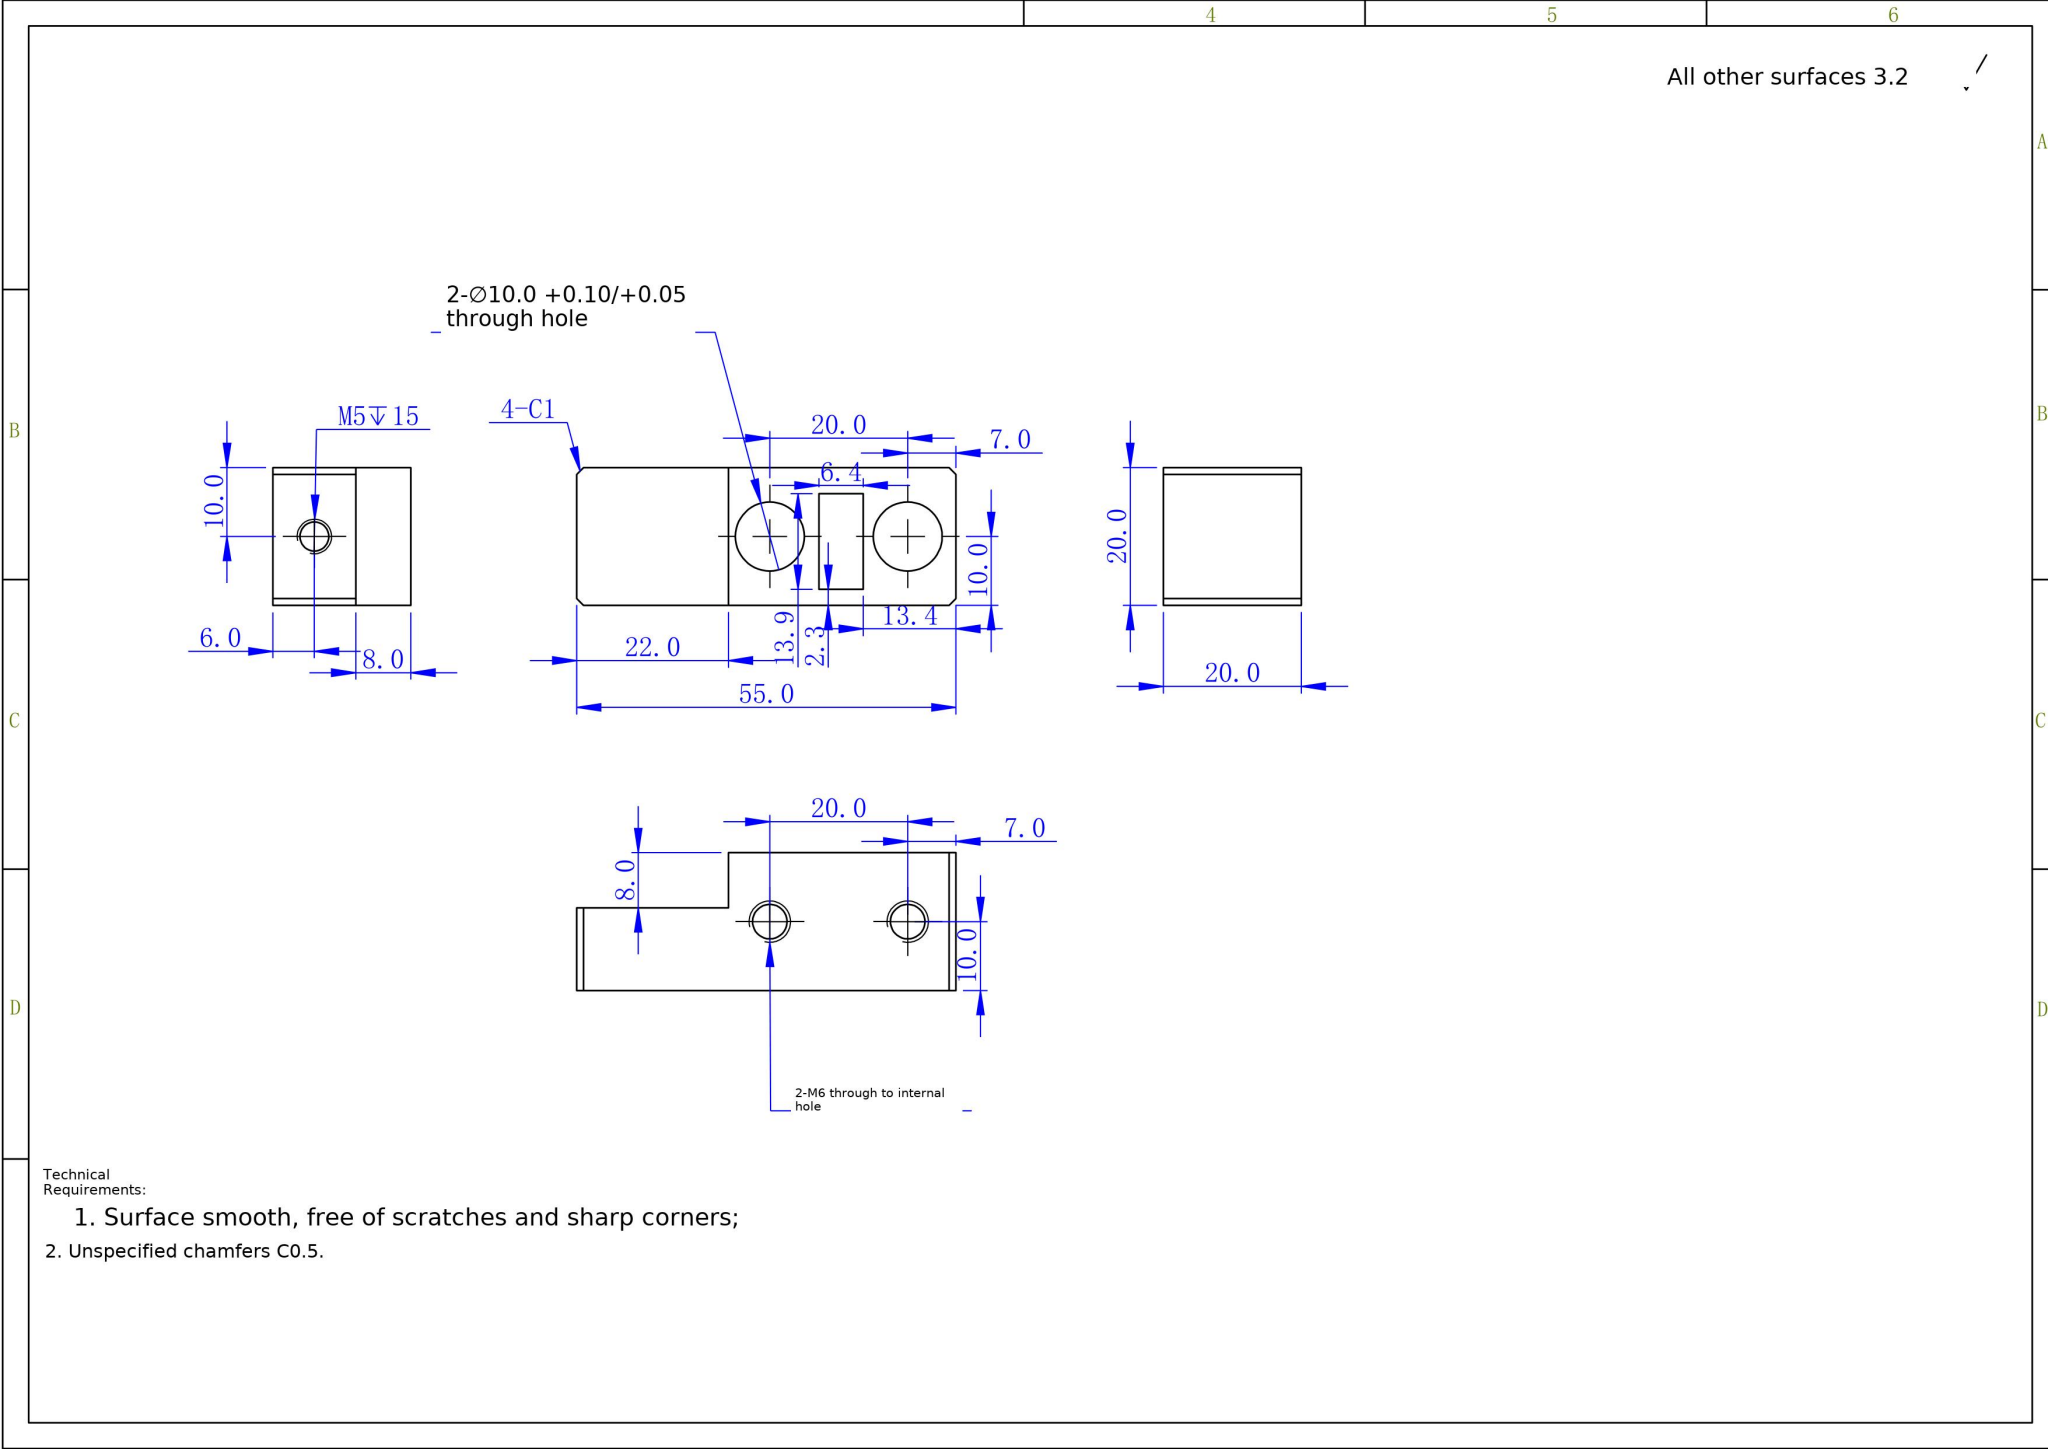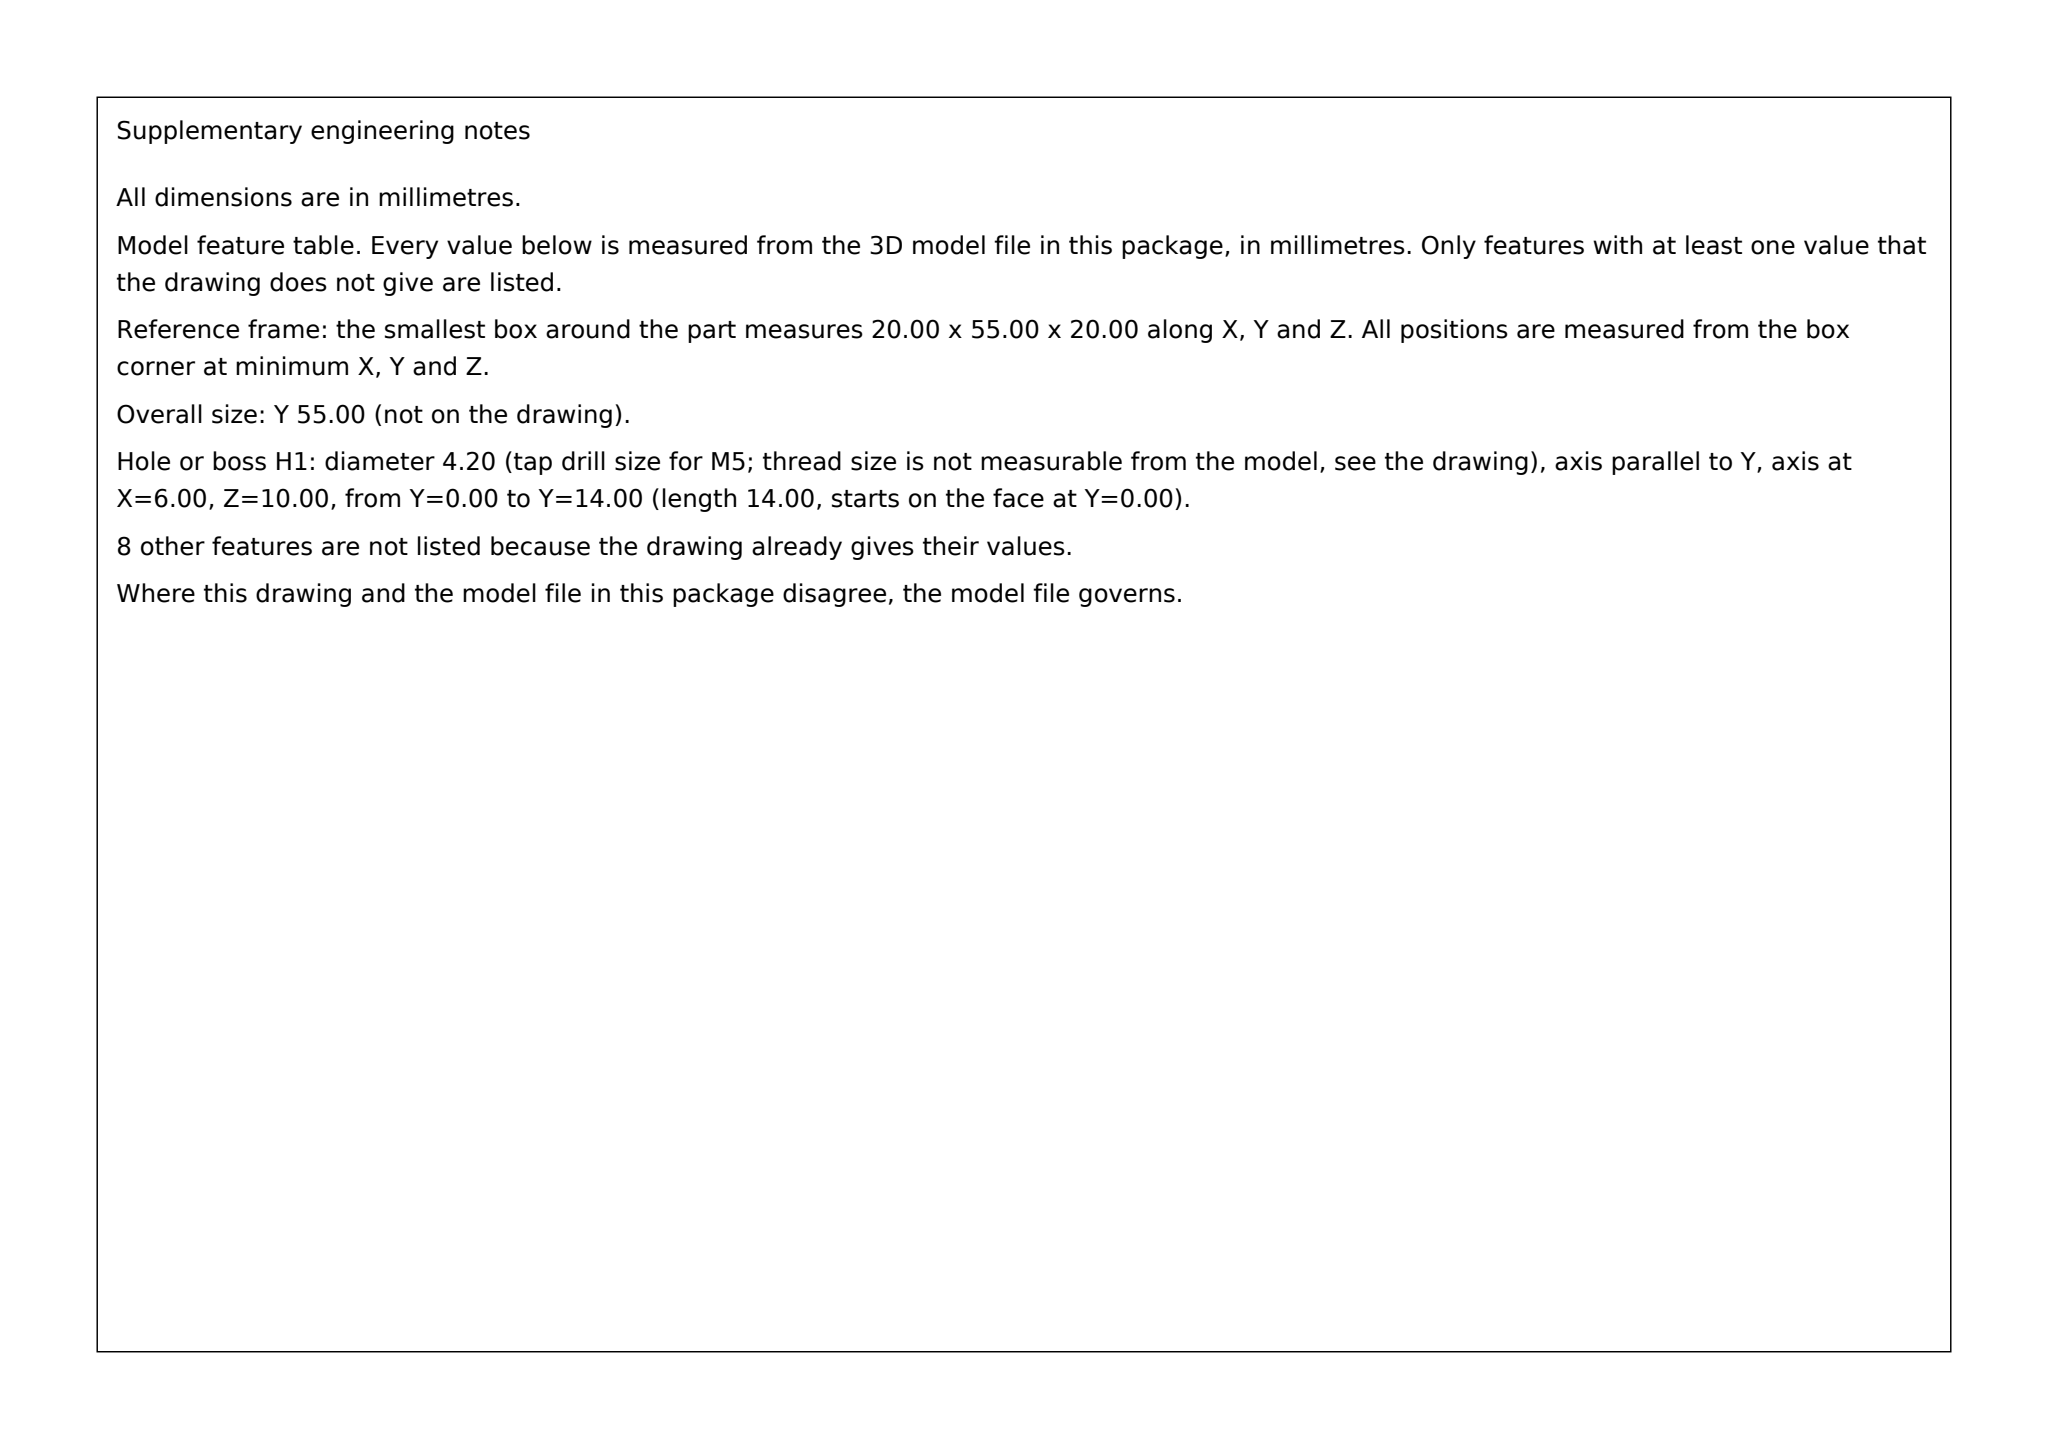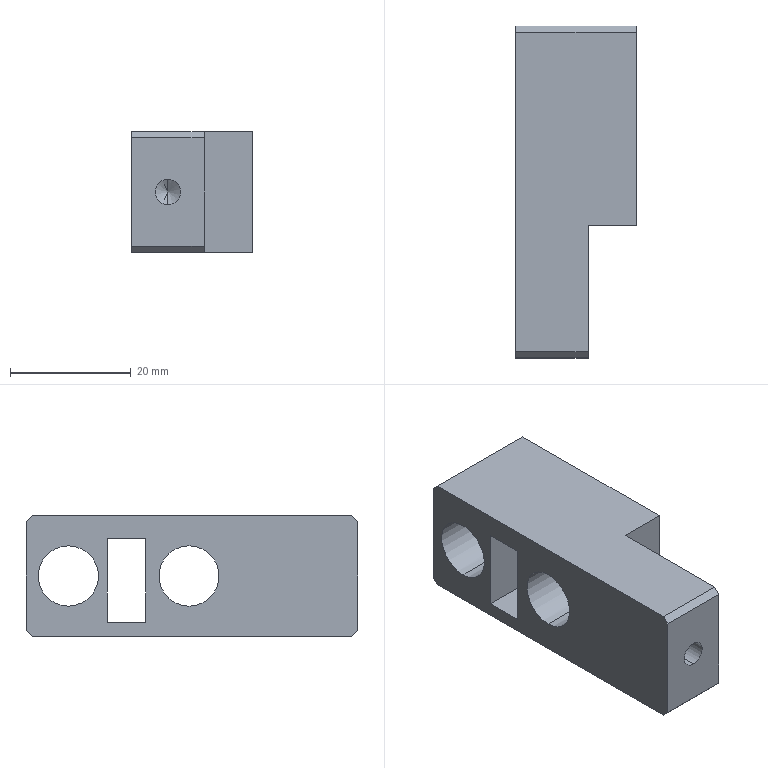Part | SolidWorks | mm | 1 solid | 28 faces | box 20 x 55 x 20 mm | volume 13125 mm3 | plane 16 | cylinder 10 | cone 2 | commonest cylinder face diameters 10 x4 5 x4 4.2 x2